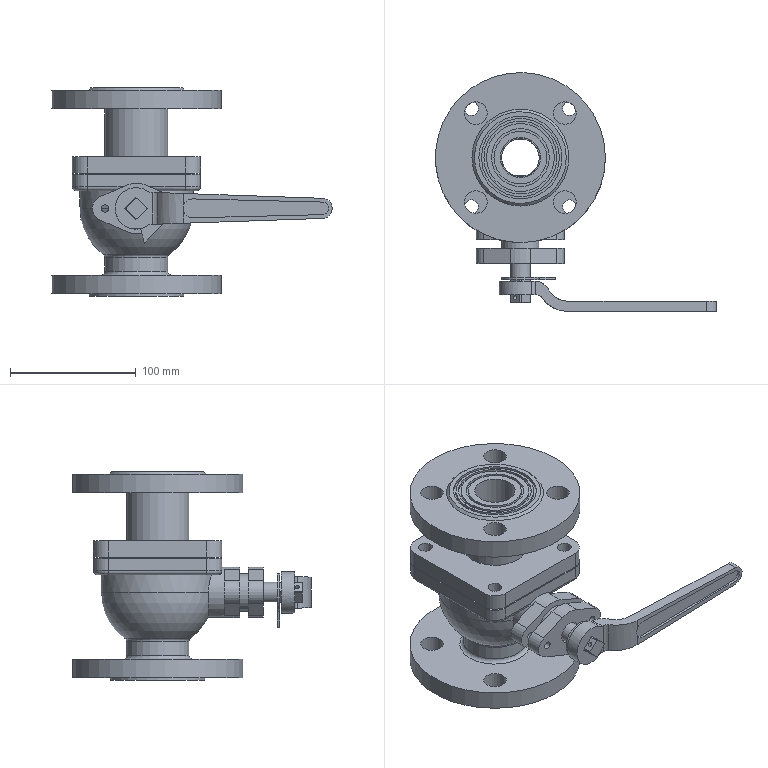Assembly | NX | mm | 10 component files | 10 solids | 215 faces | box 223.15 x 189.47 x 166 mm | volume 925175 mm3 | plane 100 | cylinder 94 | torus 8 | sphere 6 | spline 6 | cone 1 | commonest cylinder face diameters 18 x15 6 x9 24 x8 11 x8 40 x7 30 x7 10 x5 20 x4
Bill of materials:
unnamed part 1 | 1 |  | Flat lever or handle bar: a round boss with a square through-hole at one end, a joggled (stepped offset) section, then a long straight arm that tapers to a rounded end.
unnamed part 2 | 1 |  | Very thin flat annular ring (washer- or shim-like) with a narrow radial width compared to its diameter.
unnamed part 3 | 1 |  | Hollow housing: a bowl-shaped central body with a square four-bolt flange on top, a short neck down to a round four-bolt flange at the bottom, and a side port ending in a two-hole oval flange.
unnamed part 4 | 1 |  | Stepped shaft or spindle: a cylindrical main body with a larger-diameter collar near one end and flat-sided (square-section) ends at both ends.
unnamed part 5 | 1 |  | Flanged spool or adapter: a round four-hole flange and a square four-hole flange joined by a cylindrical neck, with a central through-bore.
unnamed part 6 | 1 |  | Truncated sphere with a large cylindrical through-bore between its flat ends and an oblong (obround) slot cut into one side.
unnamed part 7 | 1 |  | Thin flat plate made of a circular disc with a square through-hole and an attached triangular or flared tab, like a pointer.
unnamed part 8 | 2 |  | Plain flat annular ring with a rectangular cross-section, thicker than a shim, with moderate radial width.
unnamed part 9 | 1 |  | Two-hole flanged spigot: a diamond/oval flange with two bolt holes and a cylindrical boss projecting from one face, with a central through-bore.
Mates:
1. fix | valve_body 1 component
2. concentric | valve_core 1 edge | valve_body 1 edge
3. touch align | valve_stem 1 edge | valve_body 1 edge
4. touch align | valve_core 1 face | valve_stem 1 face
5. concentric | core_seal 2 edge | valve_body 1 edge
6. touch align | gland 1 face | valve_body 1 edge
7. touch align | gland 1 face | valve_body 1 face
8. concentric | gland 1 edge | valve_body 1 edge
9. concentric | limit_plate 1 edge | valve_stem 1 edge
10. touch align | limit_plate 1 face | valve_stem 1 face
11. touch align | wrench 1 face | valve_stem 1 face
12. concentric | bonnet_gasket 1 edge | valve_body 1 edge
13. concentric | valve_bonnet 1 edge | bonnet_gasket 1 edge
14. touch align | valve_bonnet 1 face | valve_body 1 face